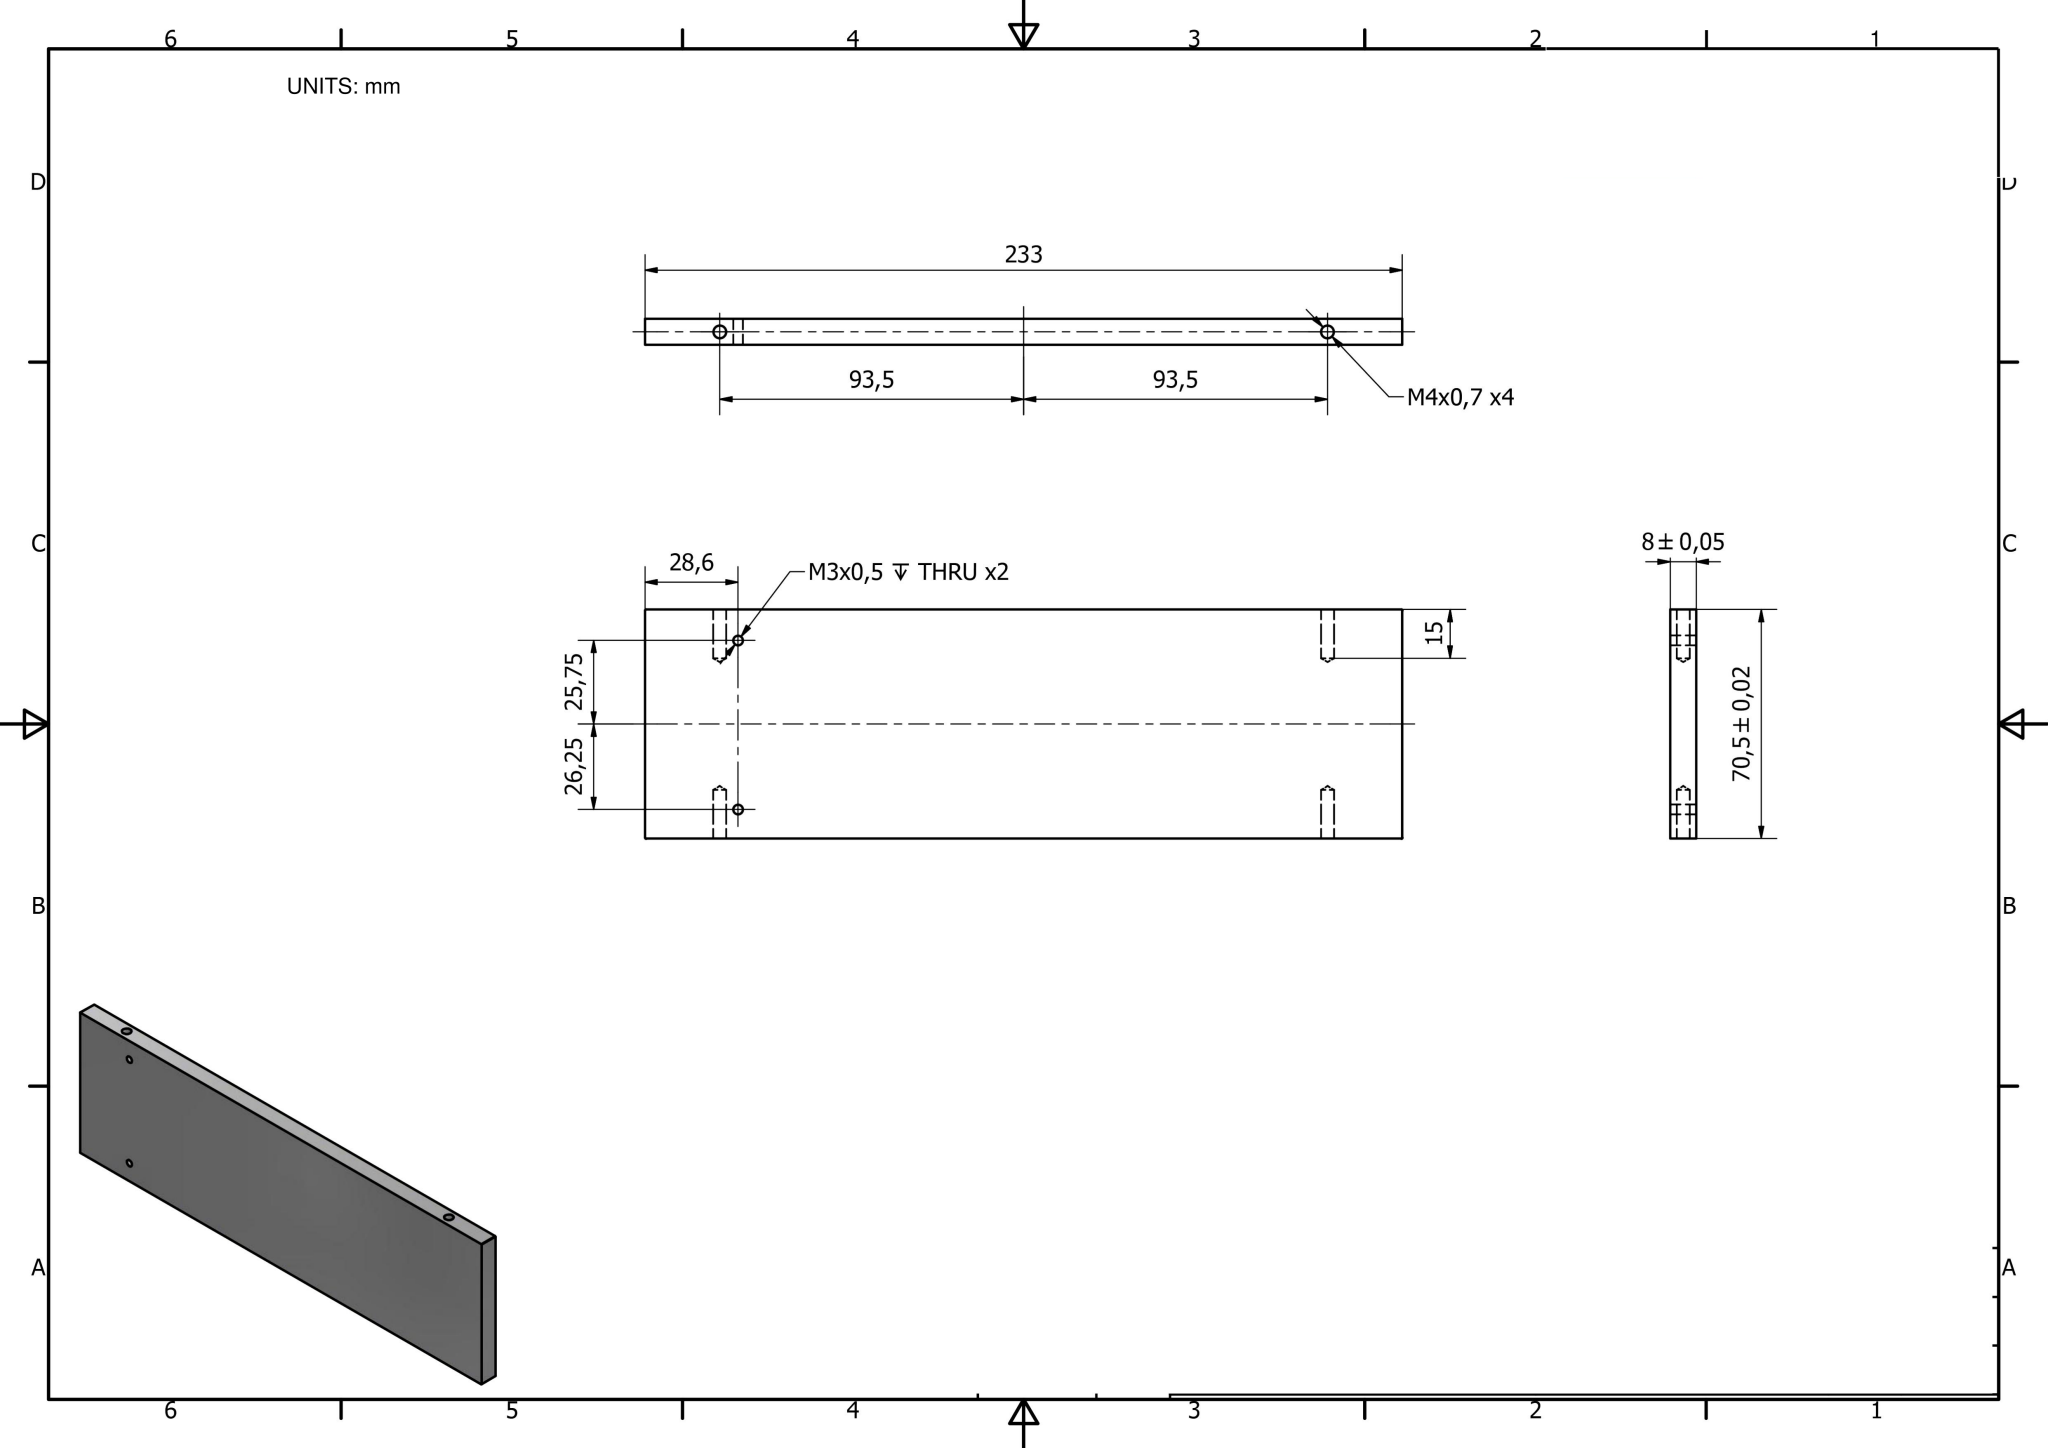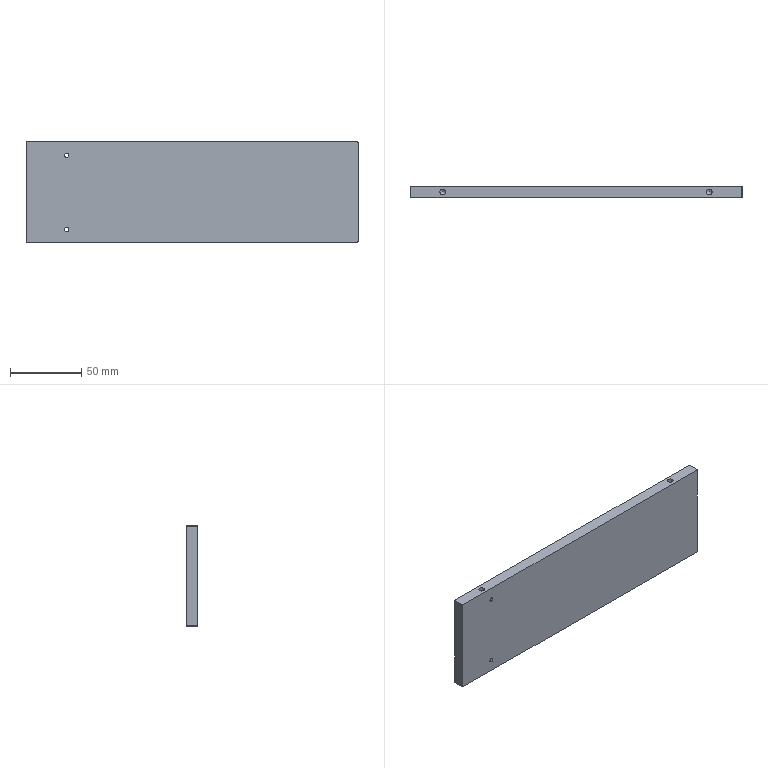Part | NX | mm | 1 solid | 20 faces | box 233 x 8 x 70.5 mm | volume 130524 mm3 | cylinder 10 | plane 6 | cone 4 | commonest cylinder face diameters 0.6 x4 4 x4 3 x2
STEP:
#1=DRAUGHTING_PRE_DEFINED_CURVE_FONT('');
#2=COLOUR_RGB('',0.9412,0.6275,0.4314);
#3=CURVE_STYLE('',#1,POSITIVE_LENGTH_MEASURE(0.000001),#2);
#4=PRESENTATION_STYLE_ASSIGNMENT((#3));
#5=CARTESIAN_POINT('',(389.001,-8.65,29.5));
#6=VERTEX_POINT('',#5);
#7=CARTESIAN_POINT('',(389.001,-6.65,29.5));
#8=DIRECTION('',(0.,0.,1.));
#9=DIRECTION('',(0.,1.,0.));
#10=AXIS2_PLACEMENT_3D('',#7,#8,#9);
#11=CIRCLE('',#10,2.);
#12=EDGE_CURVE('',#6,#6,#11,.T.);
#13=STYLED_ITEM('',(#4),#12);
#14=DRAUGHTING_PRE_DEFINED_CURVE_FONT('');
#15=COLOUR_RGB('',0.9412,0.6275,0.4314);
#16=CURVE_STYLE('',#14,POSITIVE_LENGTH_MEASURE(0.000001),#15);
#17=PRESENTATION_STYLE_ASSIGNMENT((#16));
#18=CARTESIAN_POINT('',(411.701,-10.65,29.5));
#19=VERTEX_POINT('',#18);
#20=CARTESIAN_POINT('',(411.701,-2.65,29.5));
#21=VERTEX_POINT('',#20);
#22=CARTESIAN_POINT('',(411.701,-10.65,29.5));
#23=DIRECTION('',(0.,1.,0.));
#24=VECTOR('',#23,1.);
#25=LINE('',#22,#24);
#26=EDGE_CURVE('',#19,#21,#25,.T.);
#27=STYLED_ITEM('',(#17),#26);
#28=COLOUR_RGB('',0.9412,0.6275,0.4314);
#29=FILL_AREA_STYLE_COLOUR('',#28);
#30=FILL_AREA_STYLE('',(#29));
#31=SURFACE_STYLE_FILL_AREA(#30);
#32=SURFACE_SIDE_STYLE('',(#31));
#33=SURFACE_STYLE_USAGE(.BOTH.,#32);
#34=PRESENTATION_STYLE_ASSIGNMENT((#33));
#35=CARTESIAN_POINT('',(412.001,-2.65,99.7));
#36=VERTEX_POINT('',#35);
#37=CARTESIAN_POINT('',(411.701,-2.65,100.));
#38=VERTEX_POINT('',#37);
#39=CARTESIAN_POINT('',(411.701,-2.65,99.7));
#40=DIRECTION('',(-0.,-1.,0.));
#41=DIRECTION('',(0.7071,0.,0.7071));
#42=AXIS2_PLACEMENT_3D('',#39,#40,#41);
#43=CIRCLE('',#42,0.3);
#44=EDGE_CURVE('',#36,#38,#43,.T.);
#45=ORIENTED_EDGE('',*,*,#44,.T.);
#46=CARTESIAN_POINT('',(411.701,-10.65,100.));
#47=VERTEX_POINT('',#46);
#48=CARTESIAN_POINT('',(411.701,-10.65,100.));
#49=DIRECTION('',(0.,-1.,0.));
#50=VECTOR('',#49,1.);
#51=LINE('',#48,#50);
#52=EDGE_CURVE('',#38,#47,#51,.T.);
#53=ORIENTED_EDGE('',*,*,#52,.T.);
#54=CARTESIAN_POINT('',(412.001,-10.65,99.7));
#55=VERTEX_POINT('',#54);
#56=CARTESIAN_POINT('',(411.701,-10.65,99.7));
#57=DIRECTION('',(0.,1.,-0.));
#58=DIRECTION('',(0.7071,0.,0.7071));
#59=AXIS2_PLACEMENT_3D('',#56,#57,#58);
#60=CIRCLE('',#59,0.3);
#61=EDGE_CURVE('',#47,#55,#60,.T.);
#62=ORIENTED_EDGE('',*,*,#61,.T.);
#63=CARTESIAN_POINT('',(412.001,-10.65,99.7));
#64=DIRECTION('',(0.,1.,0.));
#65=VECTOR('',#64,1.);
#66=LINE('',#63,#65);
#67=EDGE_CURVE('',#55,#36,#66,.T.);
#68=ORIENTED_EDGE('',*,*,#67,.T.);
#69=EDGE_LOOP('',(#45,#53,#62,#68));
#70=FACE_OUTER_BOUND('',#69,.T.);
#71=CARTESIAN_POINT('',(411.701,-10.65,99.7));
#72=DIRECTION('',(0.,1.,0.));
#73=DIRECTION('',(0.7071,0.,0.7071));
#74=AXIS2_PLACEMENT_3D('',#71,#72,#73);
#75=CYLINDRICAL_SURFACE('',#74,0.3);
#76=ADVANCED_FACE('',(#70),#75,.T.);
#77=CARTESIAN_POINT('',(207.601,-10.65,89.));
#78=VERTEX_POINT('',#77);
#79=CARTESIAN_POINT('',(207.601,-10.65,90.5));
#80=DIRECTION('',(-0.,-1.,0.));
#81=DIRECTION('',(0.,0.,1.));
#82=AXIS2_PLACEMENT_3D('',#79,#80,#81);
#83=CIRCLE('',#82,1.5);
#84=EDGE_CURVE('',#78,#78,#83,.F.);
#85=ORIENTED_EDGE('',*,*,#84,.T.);
#86=EDGE_LOOP('',(#85));
#87=FACE_BOUND('',#86,.T.);
#88=CARTESIAN_POINT('',(207.601,-10.65,37.));
#89=VERTEX_POINT('',#88);
#90=CARTESIAN_POINT('',(207.601,-10.65,38.5));
#91=DIRECTION('',(-0.,-1.,0.));
#92=DIRECTION('',(0.,0.,1.));
#93=AXIS2_PLACEMENT_3D('',#90,#91,#92);
#94=CIRCLE('',#93,1.5);
#95=EDGE_CURVE('',#89,#89,#94,.F.);
#96=ORIENTED_EDGE('',*,*,#95,.T.);
#97=EDGE_LOOP('',(#96));
#98=FACE_BOUND('',#97,.T.);
#99=ORIENTED_EDGE('',*,*,#61,.F.);
#100=CARTESIAN_POINT('',(179.301,-10.65,100.));
#101=VERTEX_POINT('',#100);
#102=CARTESIAN_POINT('',(179.001,-10.65,100.));
#103=DIRECTION('',(1.,0.,-0.));
#104=VECTOR('',#103,1.);
#105=LINE('',#102,#104);
#106=EDGE_CURVE('',#101,#47,#105,.T.);
#107=ORIENTED_EDGE('',*,*,#106,.F.);
#108=CARTESIAN_POINT('',(179.001,-10.65,99.7));
#109=VERTEX_POINT('',#108);
#110=CARTESIAN_POINT('',(179.301,-10.65,99.7));
#111=DIRECTION('',(0.,1.,-0.));
#112=DIRECTION('',(-0.7071,0.,0.7071));
#113=AXIS2_PLACEMENT_3D('',#110,#111,#112);
#114=CIRCLE('',#113,0.3);
#115=EDGE_CURVE('',#109,#101,#114,.T.);
#116=ORIENTED_EDGE('',*,*,#115,.F.);
#117=CARTESIAN_POINT('',(179.001,-10.65,29.8));
#118=VERTEX_POINT('',#117);
#119=CARTESIAN_POINT('',(179.001,-10.65,29.5));
#120=DIRECTION('',(0.,0.,1.));
#121=VECTOR('',#120,1.);
#122=LINE('',#119,#121);
#123=EDGE_CURVE('',#118,#109,#122,.T.);
#124=ORIENTED_EDGE('',*,*,#123,.F.);
#125=CARTESIAN_POINT('',(179.301,-10.65,29.5));
#126=VERTEX_POINT('',#125);
#127=CARTESIAN_POINT('',(179.301,-10.65,29.8));
#128=DIRECTION('',(0.,1.,-0.));
#129=DIRECTION('',(-0.7071,-0.,-0.7071));
#130=AXIS2_PLACEMENT_3D('',#127,#128,#129);
#131=CIRCLE('',#130,0.3);
#132=EDGE_CURVE('',#126,#118,#131,.T.);
#133=ORIENTED_EDGE('',*,*,#132,.F.);
#134=CARTESIAN_POINT('',(425.001,-10.65,29.5));
#135=DIRECTION('',(-1.,0.,0.));
#136=VECTOR('',#135,1.);
#137=LINE('',#134,#136);
#138=EDGE_CURVE('',#19,#126,#137,.T.);
#139=ORIENTED_EDGE('',*,*,#138,.F.);
#140=CARTESIAN_POINT('',(412.001,-10.65,29.8));
#141=VERTEX_POINT('',#140);
#142=CARTESIAN_POINT('',(411.701,-10.65,29.8));
#143=DIRECTION('',(0.,1.,-0.));
#144=DIRECTION('',(0.7071,-0.,-0.7071));
#145=AXIS2_PLACEMENT_3D('',#142,#143,#144);
#146=CIRCLE('',#145,0.3);
#147=EDGE_CURVE('',#141,#19,#146,.T.);
#148=ORIENTED_EDGE('',*,*,#147,.F.);
#149=CARTESIAN_POINT('',(412.001,-10.65,64.75));
#150=DIRECTION('',(0.,0.,1.));
#151=VECTOR('',#150,1.);
#152=LINE('',#149,#151);
#153=EDGE_CURVE('',#55,#141,#152,.F.);
#154=ORIENTED_EDGE('',*,*,#153,.F.);
#155=EDGE_LOOP('',(#99,#107,#116,#124,#133,#139,#148,#154));
#156=FACE_OUTER_BOUND('',#155,.T.);
#157=CARTESIAN_POINT('',(302.001,-10.65,64.75));
#158=DIRECTION('',(0.,1.,-0.));
#159=DIRECTION('',(0.,0.,1.));
#160=AXIS2_PLACEMENT_3D('',#157,#158,#159);
#161=PLANE('',#160);
#162=ADVANCED_FACE('',(#87,#98,#156),#161,.F.);
#163=CARTESIAN_POINT('',(389.001,-4.65,100.));
#164=VERTEX_POINT('',#163);
#165=CARTESIAN_POINT('',(389.001,-6.65,100.));
#166=DIRECTION('',(-0.,0.,-1.));
#167=DIRECTION('',(0.,-1.,0.));
#168=AXIS2_PLACEMENT_3D('',#165,#166,#167);
#169=CIRCLE('',#168,2.);
#170=EDGE_CURVE('',#164,#164,#169,.T.);
#171=ORIENTED_EDGE('',*,*,#170,.T.);
#172=EDGE_LOOP('',(#171));
#173=FACE_BOUND('',#172,.T.);
#174=CARTESIAN_POINT('',(202.001,-4.65,100.));
#175=VERTEX_POINT('',#174);
#176=CARTESIAN_POINT('',(202.001,-6.65,100.));
#177=DIRECTION('',(-0.,0.,-1.));
#178=DIRECTION('',(0.,-1.,0.));
#179=AXIS2_PLACEMENT_3D('',#176,#177,#178);
#180=CIRCLE('',#179,2.);
#181=EDGE_CURVE('',#175,#175,#180,.T.);
#182=ORIENTED_EDGE('',*,*,#181,.T.);
#183=EDGE_LOOP('',(#182));
#184=FACE_BOUND('',#183,.T.);
#185=ORIENTED_EDGE('',*,*,#52,.F.);
#186=CARTESIAN_POINT('',(179.301,-2.65,100.));
#187=VERTEX_POINT('',#186);
#188=CARTESIAN_POINT('',(179.001,-2.65,100.));
#189=DIRECTION('',(-1.,0.,0.));
#190=VECTOR('',#189,1.);
#191=LINE('',#188,#190);
#192=EDGE_CURVE('',#38,#187,#191,.T.);
#193=ORIENTED_EDGE('',*,*,#192,.T.);
#194=CARTESIAN_POINT('',(179.301,-10.65,100.));
#195=DIRECTION('',(0.,1.,0.));
#196=VECTOR('',#195,1.);
#197=LINE('',#194,#196);
#198=EDGE_CURVE('',#101,#187,#197,.T.);
#199=ORIENTED_EDGE('',*,*,#198,.F.);
#200=ORIENTED_EDGE('',*,*,#106,.T.);
#201=EDGE_LOOP('',(#185,#193,#199,#200));
#202=FACE_OUTER_BOUND('',#201,.T.);
#203=CARTESIAN_POINT('',(302.001,-10.65,100.));
#204=DIRECTION('',(0.,0.,1.));
#205=DIRECTION('',(1.,0.,-0.));
#206=AXIS2_PLACEMENT_3D('',#203,#204,#205);
#207=PLANE('',#206);
#208=ADVANCED_FACE('',(#173,#184,#202),#207,.T.);
#209=CARTESIAN_POINT('',(179.001,-2.65,99.7));
#210=VERTEX_POINT('',#209);
#211=CARTESIAN_POINT('',(179.301,-2.65,99.7));
#212=DIRECTION('',(-0.,-1.,0.));
#213=DIRECTION('',(-0.7071,0.,0.7071));
#214=AXIS2_PLACEMENT_3D('',#211,#212,#213);
#215=CIRCLE('',#214,0.3);
#216=EDGE_CURVE('',#187,#210,#215,.T.);
#217=ORIENTED_EDGE('',*,*,#216,.T.);
#218=CARTESIAN_POINT('',(179.001,-10.65,99.7));
#219=DIRECTION('',(0.,-1.,0.));
#220=VECTOR('',#219,1.);
#221=LINE('',#218,#220);
#222=EDGE_CURVE('',#210,#109,#221,.T.);
#223=ORIENTED_EDGE('',*,*,#222,.T.);
#224=ORIENTED_EDGE('',*,*,#115,.T.);
#225=ORIENTED_EDGE('',*,*,#198,.T.);
#226=EDGE_LOOP('',(#217,#223,#224,#225));
#227=FACE_OUTER_BOUND('',#226,.T.);
#228=CARTESIAN_POINT('',(179.301,-10.65,99.7));
#229=DIRECTION('',(0.,1.,0.));
#230=DIRECTION('',(-0.7071,0.,0.7071));
#231=AXIS2_PLACEMENT_3D('',#228,#229,#230);
#232=CYLINDRICAL_SURFACE('',#231,0.3);
#233=ADVANCED_FACE('',(#227),#232,.T.);
#234=CARTESIAN_POINT('',(412.001,-2.65,29.8));
#235=VERTEX_POINT('',#234);
#236=CARTESIAN_POINT('',(411.701,-2.65,29.8));
#237=DIRECTION('',(-0.,-1.,0.));
#238=DIRECTION('',(0.7071,-0.,-0.7071));
#239=AXIS2_PLACEMENT_3D('',#236,#237,#238);
#240=CIRCLE('',#239,0.3);
#241=EDGE_CURVE('',#21,#235,#240,.T.);
#242=ORIENTED_EDGE('',*,*,#241,.T.);
#243=CARTESIAN_POINT('',(412.001,-10.65,29.8));
#244=DIRECTION('',(0.,-1.,0.));
#245=VECTOR('',#244,1.);
#246=LINE('',#243,#245);
#247=EDGE_CURVE('',#235,#141,#246,.T.);
#248=ORIENTED_EDGE('',*,*,#247,.T.);
#249=ORIENTED_EDGE('',*,*,#147,.T.);
#250=ORIENTED_EDGE('',*,*,#26,.T.);
#251=EDGE_LOOP('',(#242,#248,#249,#250));
#252=FACE_OUTER_BOUND('',#251,.T.);
#253=CARTESIAN_POINT('',(411.701,-10.65,29.8));
#254=DIRECTION('',(0.,1.,0.));
#255=DIRECTION('',(0.7071,0.,-0.7071));
#256=AXIS2_PLACEMENT_3D('',#253,#254,#255);
#257=CYLINDRICAL_SURFACE('',#256,0.3);
#258=ADVANCED_FACE('',(#252),#257,.T.);
#259=CARTESIAN_POINT('',(202.001,-8.65,29.5));
#260=VERTEX_POINT('',#259);
#261=CARTESIAN_POINT('',(202.001,-6.65,29.5));
#262=DIRECTION('',(0.,0.,1.));
#263=DIRECTION('',(0.,1.,0.));
#264=AXIS2_PLACEMENT_3D('',#261,#262,#263);
#265=CIRCLE('',#264,2.);
#266=EDGE_CURVE('',#260,#260,#265,.T.);
#267=ORIENTED_EDGE('',*,*,#266,.T.);
#268=EDGE_LOOP('',(#267));
#269=FACE_BOUND('',#268,.T.);
#270=ORIENTED_EDGE('',*,*,#12,.T.);
#271=EDGE_LOOP('',(#270));
#272=FACE_BOUND('',#271,.T.);
#273=ORIENTED_EDGE('',*,*,#26,.F.);
#274=ORIENTED_EDGE('',*,*,#138,.T.);
#275=CARTESIAN_POINT('',(179.301,-2.65,29.5));
#276=VERTEX_POINT('',#275);
#277=CARTESIAN_POINT('',(179.301,-10.65,29.5));
#278=DIRECTION('',(0.,-1.,0.));
#279=VECTOR('',#278,1.);
#280=LINE('',#277,#279);
#281=EDGE_CURVE('',#276,#126,#280,.T.);
#282=ORIENTED_EDGE('',*,*,#281,.F.);
#283=CARTESIAN_POINT('',(425.001,-2.65,29.5));
#284=DIRECTION('',(1.,0.,-0.));
#285=VECTOR('',#284,1.);
#286=LINE('',#283,#285);
#287=EDGE_CURVE('',#276,#21,#286,.T.);
#288=ORIENTED_EDGE('',*,*,#287,.T.);
#289=EDGE_LOOP('',(#273,#274,#282,#288));
#290=FACE_OUTER_BOUND('',#289,.T.);
#291=CARTESIAN_POINT('',(302.001,-10.65,29.5));
#292=DIRECTION('',(-0.,0.,-1.));
#293=DIRECTION('',(-1.,0.,0.));
#294=AXIS2_PLACEMENT_3D('',#291,#292,#293);
#295=PLANE('',#294);
#296=ADVANCED_FACE('',(#269,#272,#290),#295,.T.);
#297=CARTESIAN_POINT('',(179.001,-2.65,29.8));
#298=VERTEX_POINT('',#297);
#299=CARTESIAN_POINT('',(179.301,-2.65,29.8));
#300=DIRECTION('',(-0.,-1.,0.));
#301=DIRECTION('',(-0.7071,-0.,-0.7071));
#302=AXIS2_PLACEMENT_3D('',#299,#300,#301);
#303=CIRCLE('',#302,0.3);
#304=EDGE_CURVE('',#298,#276,#303,.T.);
#305=ORIENTED_EDGE('',*,*,#304,.T.);
#306=ORIENTED_EDGE('',*,*,#281,.T.);
#307=ORIENTED_EDGE('',*,*,#132,.T.);
#308=CARTESIAN_POINT('',(179.001,-10.65,29.8));
#309=DIRECTION('',(0.,1.,0.));
#310=VECTOR('',#309,1.);
#311=LINE('',#308,#310);
#312=EDGE_CURVE('',#118,#298,#311,.T.);
#313=ORIENTED_EDGE('',*,*,#312,.T.);
#314=EDGE_LOOP('',(#305,#306,#307,#313));
#315=FACE_OUTER_BOUND('',#314,.T.);
#316=CARTESIAN_POINT('',(179.301,-10.65,29.8));
#317=DIRECTION('',(0.,1.,0.));
#318=DIRECTION('',(-0.7071,0.,-0.7071));
#319=AXIS2_PLACEMENT_3D('',#316,#317,#318);
#320=CYLINDRICAL_SURFACE('',#319,0.3);
#321=ADVANCED_FACE('',(#315),#320,.T.);
#322=ORIENTED_EDGE('',*,*,#67,.F.);
#323=ORIENTED_EDGE('',*,*,#153,.T.);
#324=ORIENTED_EDGE('',*,*,#247,.F.);
#325=CARTESIAN_POINT('',(412.001,-2.65,64.75));
#326=DIRECTION('',(0.,0.,1.));
#327=VECTOR('',#326,1.);
#328=LINE('',#325,#327);
#329=EDGE_CURVE('',#235,#36,#328,.T.);
#330=ORIENTED_EDGE('',*,*,#329,.T.);
#331=EDGE_LOOP('',(#322,#323,#324,#330));
#332=FACE_OUTER_BOUND('',#331,.T.);
#333=CARTESIAN_POINT('',(412.001,-10.65,64.75));
#334=DIRECTION('',(1.,0.,0.));
#335=DIRECTION('',(0.,0.,-1.));
#336=AXIS2_PLACEMENT_3D('',#333,#334,#335);
#337=PLANE('',#336);
#338=ADVANCED_FACE('',(#332),#337,.T.);
#339=ORIENTED_EDGE('',*,*,#44,.F.);
#340=ORIENTED_EDGE('',*,*,#329,.F.);
#341=ORIENTED_EDGE('',*,*,#241,.F.);
#342=ORIENTED_EDGE('',*,*,#287,.F.);
#343=ORIENTED_EDGE('',*,*,#304,.F.);
#344=CARTESIAN_POINT('',(179.001,-2.65,29.5));
#345=DIRECTION('',(0.,0.,-1.));
#346=VECTOR('',#345,1.);
#347=LINE('',#344,#346);
#348=EDGE_CURVE('',#210,#298,#347,.T.);
#349=ORIENTED_EDGE('',*,*,#348,.F.);
#350=ORIENTED_EDGE('',*,*,#216,.F.);
#351=ORIENTED_EDGE('',*,*,#192,.F.);
#352=EDGE_LOOP('',(#339,#340,#341,#342,#343,#349,#350,#351));
#353=FACE_OUTER_BOUND('',#352,.T.);
#354=CARTESIAN_POINT('',(207.601,-2.65,89.));
#355=VERTEX_POINT('',#354);
#356=CARTESIAN_POINT('',(207.601,-2.65,90.5));
#357=DIRECTION('',(-0.,-1.,0.));
#358=DIRECTION('',(0.,0.,1.));
#359=AXIS2_PLACEMENT_3D('',#356,#357,#358);
#360=CIRCLE('',#359,1.5);
#361=EDGE_CURVE('',#355,#355,#360,.T.);
#362=ORIENTED_EDGE('',*,*,#361,.T.);
#363=EDGE_LOOP('',(#362));
#364=FACE_BOUND('',#363,.T.);
#365=CARTESIAN_POINT('',(207.601,-2.65,37.));
#366=VERTEX_POINT('',#365);
#367=CARTESIAN_POINT('',(207.601,-2.65,38.5));
#368=DIRECTION('',(-0.,-1.,0.));
#369=DIRECTION('',(0.,0.,1.));
#370=AXIS2_PLACEMENT_3D('',#367,#368,#369);
#371=CIRCLE('',#370,1.5);
#372=EDGE_CURVE('',#366,#366,#371,.T.);
#373=ORIENTED_EDGE('',*,*,#372,.T.);
#374=EDGE_LOOP('',(#373));
#375=FACE_BOUND('',#374,.T.);
#376=CARTESIAN_POINT('',(302.001,-2.65,64.75));
#377=DIRECTION('',(0.,1.,-0.));
#378=DIRECTION('',(0.,0.,1.));
#379=AXIS2_PLACEMENT_3D('',#376,#377,#378);
#380=PLANE('',#379);
#381=ADVANCED_FACE('',(#353,#364,#375),#380,.T.);
#382=CARTESIAN_POINT('',(389.001,-8.65,85.));
#383=VERTEX_POINT('',#382);
#384=CARTESIAN_POINT('',(389.001,-6.65,85.));
#385=DIRECTION('',(0.,0.,1.));
#386=DIRECTION('',(0.,-1.,0.));
#387=AXIS2_PLACEMENT_3D('',#384,#385,#386);
#388=CIRCLE('',#387,2.);
#389=EDGE_CURVE('',#383,#383,#388,.T.);
#390=ORIENTED_EDGE('',*,*,#389,.T.);
#391=EDGE_LOOP('',(#390));
#392=FACE_BOUND('',#391,.T.);
#393=CARTESIAN_POINT('',(389.001,-6.65,83.798));
#394=VERTEX_POINT('',#393);
#395=VERTEX_LOOP('',#394);
#396=FACE_BOUND('',#395,.T.);
#397=CARTESIAN_POINT('',(389.001,-6.65,84.399));
#398=DIRECTION('',(0.,0.,1.));
#399=DIRECTION('',(1.,0.,0.));
#400=AXIS2_PLACEMENT_3D('',#397,#398,#399);
#401=CONICAL_SURFACE('',#400,1.,1.03);
#402=ADVANCED_FACE('',(#392,#396),#401,.F.);
#403=ORIENTED_EDGE('',*,*,#170,.F.);
#404=EDGE_LOOP('',(#403));
#405=FACE_BOUND('',#404,.T.);
#406=ORIENTED_EDGE('',*,*,#389,.F.);
#407=EDGE_LOOP('',(#406));
#408=FACE_BOUND('',#407,.T.);
#409=CARTESIAN_POINT('',(389.001,-6.65,104.));
#410=DIRECTION('',(0.,0.,-1.));
#411=DIRECTION('',(0.,-1.,0.));
#412=AXIS2_PLACEMENT_3D('',#409,#410,#411);
#413=CYLINDRICAL_SURFACE('',#412,2.);
#414=ADVANCED_FACE('',(#405,#408),#413,.F.);
#415=CARTESIAN_POINT('',(202.001,-8.65,85.));
#416=VERTEX_POINT('',#415);
#417=CARTESIAN_POINT('',(202.001,-6.65,85.));
#418=DIRECTION('',(0.,0.,1.));
#419=DIRECTION('',(0.,-1.,0.));
#420=AXIS2_PLACEMENT_3D('',#417,#418,#419);
#421=CIRCLE('',#420,2.);
#422=EDGE_CURVE('',#416,#416,#421,.T.);
#423=ORIENTED_EDGE('',*,*,#422,.T.);
#424=EDGE_LOOP('',(#423));
#425=FACE_BOUND('',#424,.T.);
#426=CARTESIAN_POINT('',(202.001,-6.65,83.798));
#427=VERTEX_POINT('',#426);
#428=VERTEX_LOOP('',#427);
#429=FACE_BOUND('',#428,.T.);
#430=CARTESIAN_POINT('',(202.001,-6.65,84.399));
#431=DIRECTION('',(0.,0.,1.));
#432=DIRECTION('',(1.,0.,0.));
#433=AXIS2_PLACEMENT_3D('',#430,#431,#432);
#434=CONICAL_SURFACE('',#433,1.,1.03);
#435=ADVANCED_FACE('',(#425,#429),#434,.F.);
#436=ORIENTED_EDGE('',*,*,#181,.F.);
#437=EDGE_LOOP('',(#436));
#438=FACE_BOUND('',#437,.T.);
#439=ORIENTED_EDGE('',*,*,#422,.F.);
#440=EDGE_LOOP('',(#439));
#441=FACE_BOUND('',#440,.T.);
#442=CARTESIAN_POINT('',(202.001,-6.65,104.));
#443=DIRECTION('',(0.,0.,-1.));
#444=DIRECTION('',(0.,-1.,0.));
#445=AXIS2_PLACEMENT_3D('',#442,#443,#444);
#446=CYLINDRICAL_SURFACE('',#445,2.);
#447=ADVANCED_FACE('',(#438,#441),#446,.F.);
#448=CARTESIAN_POINT('',(202.001,-4.65,44.5));
#449=VERTEX_POINT('',#448);
#450=CARTESIAN_POINT('',(202.001,-6.65,44.5));
#451=DIRECTION('',(-0.,0.,-1.));
#452=DIRECTION('',(0.,1.,0.));
#453=AXIS2_PLACEMENT_3D('',#450,#451,#452);
#454=CIRCLE('',#453,2.);
#455=EDGE_CURVE('',#449,#449,#454,.T.);
#456=ORIENTED_EDGE('',*,*,#455,.T.);
#457=EDGE_LOOP('',(#456));
#458=FACE_BOUND('',#457,.T.);
#459=CARTESIAN_POINT('',(202.001,-6.65,45.702));
#460=VERTEX_POINT('',#459);
#461=VERTEX_LOOP('',#460);
#462=FACE_BOUND('',#461,.T.);
#463=CARTESIAN_POINT('',(202.001,-6.65,45.101));
#464=DIRECTION('',(0.,0.,-1.));
#465=DIRECTION('',(1.,0.,0.));
#466=AXIS2_PLACEMENT_3D('',#463,#464,#465);
#467=CONICAL_SURFACE('',#466,1.,1.03);
#468=ADVANCED_FACE('',(#458,#462),#467,.F.);
#469=ORIENTED_EDGE('',*,*,#266,.F.);
#470=EDGE_LOOP('',(#469));
#471=FACE_BOUND('',#470,.T.);
#472=ORIENTED_EDGE('',*,*,#455,.F.);
#473=EDGE_LOOP('',(#472));
#474=FACE_BOUND('',#473,.T.);
#475=CARTESIAN_POINT('',(202.001,-6.65,25.5));
#476=DIRECTION('',(0.,0.,1.));
#477=DIRECTION('',(0.,1.,0.));
#478=AXIS2_PLACEMENT_3D('',#475,#476,#477);
#479=CYLINDRICAL_SURFACE('',#478,2.);
#480=ADVANCED_FACE('',(#471,#474),#479,.F.);
#481=CARTESIAN_POINT('',(389.001,-4.65,44.5));
#482=VERTEX_POINT('',#481);
#483=CARTESIAN_POINT('',(389.001,-6.65,44.5));
#484=DIRECTION('',(-0.,0.,-1.));
#485=DIRECTION('',(0.,1.,0.));
#486=AXIS2_PLACEMENT_3D('',#483,#484,#485);
#487=CIRCLE('',#486,2.);
#488=EDGE_CURVE('',#482,#482,#487,.T.);
#489=ORIENTED_EDGE('',*,*,#488,.T.);
#490=EDGE_LOOP('',(#489));
#491=FACE_BOUND('',#490,.T.);
#492=CARTESIAN_POINT('',(389.001,-6.65,45.702));
#493=VERTEX_POINT('',#492);
#494=VERTEX_LOOP('',#493);
#495=FACE_BOUND('',#494,.T.);
#496=CARTESIAN_POINT('',(389.001,-6.65,45.101));
#497=DIRECTION('',(0.,0.,-1.));
#498=DIRECTION('',(1.,0.,0.));
#499=AXIS2_PLACEMENT_3D('',#496,#497,#498);
#500=CONICAL_SURFACE('',#499,1.,1.03);
#501=ADVANCED_FACE('',(#491,#495),#500,.F.);
#502=ORIENTED_EDGE('',*,*,#12,.F.);
#503=EDGE_LOOP('',(#502));
#504=FACE_BOUND('',#503,.T.);
#505=ORIENTED_EDGE('',*,*,#488,.F.);
#506=EDGE_LOOP('',(#505));
#507=FACE_BOUND('',#506,.T.);
#508=CARTESIAN_POINT('',(389.001,-6.65,25.5));
#509=DIRECTION('',(0.,0.,1.));
#510=DIRECTION('',(0.,1.,0.));
#511=AXIS2_PLACEMENT_3D('',#508,#509,#510);
#512=CYLINDRICAL_SURFACE('',#511,2.);
#513=ADVANCED_FACE('',(#504,#507),#512,.F.);
#514=ORIENTED_EDGE('',*,*,#84,.F.);
#515=EDGE_LOOP('',(#514));
#516=FACE_BOUND('',#515,.T.);
#517=ORIENTED_EDGE('',*,*,#361,.F.);
#518=EDGE_LOOP('',(#517));
#519=FACE_BOUND('',#518,.T.);
#520=CARTESIAN_POINT('',(207.601,0.35,90.5));
#521=DIRECTION('',(0.,-1.,0.));
#522=DIRECTION('',(0.,0.,1.));
#523=AXIS2_PLACEMENT_3D('',#520,#521,#522);
#524=CYLINDRICAL_SURFACE('',#523,1.5);
#525=ADVANCED_FACE('',(#516,#519),#524,.F.);
#526=ORIENTED_EDGE('',*,*,#95,.F.);
#527=EDGE_LOOP('',(#526));
#528=FACE_BOUND('',#527,.T.);
#529=ORIENTED_EDGE('',*,*,#372,.F.);
#530=EDGE_LOOP('',(#529));
#531=FACE_BOUND('',#530,.T.);
#532=CARTESIAN_POINT('',(207.601,0.35,38.5));
#533=DIRECTION('',(0.,-1.,0.));
#534=DIRECTION('',(0.,0.,1.));
#535=AXIS2_PLACEMENT_3D('',#532,#533,#534);
#536=CYLINDRICAL_SURFACE('',#535,1.5);
#537=ADVANCED_FACE('',(#528,#531),#536,.F.);
#538=ORIENTED_EDGE('',*,*,#222,.F.);
#539=ORIENTED_EDGE('',*,*,#348,.T.);
#540=ORIENTED_EDGE('',*,*,#312,.F.);
#541=ORIENTED_EDGE('',*,*,#123,.T.);
#542=EDGE_LOOP('',(#538,#539,#540,#541));
#543=FACE_OUTER_BOUND('',#542,.T.);
#544=CARTESIAN_POINT('',(179.001,-10.65,64.75));
#545=DIRECTION('',(-1.,0.,0.));
#546=DIRECTION('',(0.,0.,1.));
#547=AXIS2_PLACEMENT_3D('',#544,#545,#546);
#548=PLANE('',#547);
#549=ADVANCED_FACE('',(#543),#548,.T.);
#550=CLOSED_SHELL('',(#76,#162,#208,#233,#258,#296,#321,#338,#381,#402,#414,#435,#447,#468,#480,#501,#513,#525,#537,#549));
#551=MANIFOLD_SOLID_BREP('',#550);
#552=STYLED_ITEM('',(#34),#551);
#553=DRAUGHTING_PRE_DEFINED_CURVE_FONT('');
#554=COLOUR_RGB('',0.9412,0.6275,0.4314);
#555=CURVE_STYLE('',#553,POSITIVE_LENGTH_MEASURE(0.000001),#554);
#556=PRESENTATION_STYLE_ASSIGNMENT((#555));
#557=STYLED_ITEM('',(#556),#198);
#558=COLOUR_RGB('',0.9412,0.6275,0.4314);
#559=FILL_AREA_STYLE_COLOUR('',#558);
#560=FILL_AREA_STYLE('',(#559));
#561=SURFACE_STYLE_FILL_AREA(#560);
#562=SURFACE_SIDE_STYLE('',(#561));
#563=SURFACE_STYLE_USAGE(.BOTH.,#562);
#564=PRESENTATION_STYLE_ASSIGNMENT((#563));
#565=STYLED_ITEM('',(#564),#501);
#566=COLOUR_RGB('',0.9412,0.6275,0.4314);
#567=FILL_AREA_STYLE_COLOUR('',#566);
#568=FILL_AREA_STYLE('',(#567));
#569=SURFACE_STYLE_FILL_AREA(#568);
#570=SURFACE_SIDE_STYLE('',(#569));
#571=SURFACE_STYLE_USAGE(.BOTH.,#570);
#572=PRESENTATION_STYLE_ASSIGNMENT((#571));
#573=STYLED_ITEM('',(#572),#208);
#574=DRAUGHTING_PRE_DEFINED_CURVE_FONT('');
#575=COLOUR_RGB('',0.9412,0.6275,0.4314);
#576=CURVE_STYLE('',#574,POSITIVE_LENGTH_MEASURE(0.000001),#575);
#577=PRESENTATION_STYLE_ASSIGNMENT((#576));
#578=STYLED_ITEM('',(#577),#372);
#579=COLOUR_RGB('',0.9412,0.6275,0.4314);
#580=FILL_AREA_STYLE_COLOUR('',#579);
#581=FILL_AREA_STYLE('',(#580));
#582=SURFACE_STYLE_FILL_AREA(#581);
#583=SURFACE_SIDE_STYLE('',(#582));
#584=SURFACE_STYLE_USAGE(.BOTH.,#583);
#585=PRESENTATION_STYLE_ASSIGNMENT((#584));
#586=STYLED_ITEM('',(#585),#321);
#587=COLOUR_RGB('',0.9412,0.6275,0.4314);
#588=FILL_AREA_STYLE_COLOUR('',#587);
#589=FILL_AREA_STYLE('',(#588));
#590=SURFACE_STYLE_FILL_AREA(#589);
#591=SURFACE_SIDE_STYLE('',(#590));
#592=SURFACE_STYLE_USAGE(.BOTH.,#591);
#593=PRESENTATION_STYLE_ASSIGNMENT((#592));
#594=STYLED_ITEM('',(#593),#537);
#595=COLOUR_RGB('',0.9412,0.6275,0.4314);
#596=FILL_AREA_STYLE_COLOUR('',#595);
#597=FILL_AREA_STYLE('',(#596));
#598=SURFACE_STYLE_FILL_AREA(#597);
#599=SURFACE_SIDE_STYLE('',(#598));
#600=SURFACE_STYLE_USAGE(.BOTH.,#599);
#601=PRESENTATION_STYLE_ASSIGNMENT((#600));
#602=STYLED_ITEM('',(#601),#525);
#603=COLOUR_RGB('',0.9412,0.6275,0.4314);
#604=FILL_AREA_STYLE_COLOUR('',#603);
#605=FILL_AREA_STYLE('',(#604));
#606=SURFACE_STYLE_FILL_AREA(#605);
#607=SURFACE_SIDE_STYLE('',(#606));
#608=SURFACE_STYLE_USAGE(.BOTH.,#607);
#609=PRESENTATION_STYLE_ASSIGNMENT((#608));
#610=STYLED_ITEM('',(#609),#338);
#611=COLOUR_RGB('',0.9412,0.6275,0.4314);
#612=FILL_AREA_STYLE_COLOUR('',#611);
#613=FILL_AREA_STYLE('',(#612));
#614=SURFACE_STYLE_FILL_AREA(#613);
#615=SURFACE_SIDE_STYLE('',(#614));
#616=SURFACE_STYLE_USAGE(.BOTH.,#615);
#617=PRESENTATION_STYLE_ASSIGNMENT((#616));
#618=STYLED_ITEM('',(#617),#447);
#619=COLOUR_RGB('',0.9412,0.6275,0.4314);
#620=FILL_AREA_STYLE_COLOUR('',#619);
#621=FILL_AREA_STYLE('',(#620));
#622=SURFACE_STYLE_FILL_AREA(#621);
#623=SURFACE_SIDE_STYLE('',(#622));
#624=SURFACE_STYLE_USAGE(.BOTH.,#623);
#625=PRESENTATION_STYLE_ASSIGNMENT((#624));
#626=STYLED_ITEM('',(#625),#414);
#627=DRAUGHTING_PRE_DEFINED_CURVE_FONT('');
#628=COLOUR_RGB('',0.9412,0.6275,0.4314);
#629=CURVE_STYLE('',#627,POSITIVE_LENGTH_MEASURE(0.000001),#628);
#630=PRESENTATION_STYLE_ASSIGNMENT((#629));
#631=STYLED_ITEM('',(#630),#348);
#632=DRAUGHTING_PRE_DEFINED_CURVE_FONT('');
#633=COLOUR_RGB('',0.9412,0.6275,0.4314);
#634=CURVE_STYLE('',#632,POSITIVE_LENGTH_MEASURE(0.000001),#633);
#635=PRESENTATION_STYLE_ASSIGNMENT((#634));
#636=STYLED_ITEM('',(#635),#488);
#637=DRAUGHTING_PRE_DEFINED_CURVE_FONT('');
#638=COLOUR_RGB('',0.9412,0.6275,0.4314);
#639=CURVE_STYLE('',#637,POSITIVE_LENGTH_MEASURE(0.000001),#638);
#640=PRESENTATION_STYLE_ASSIGNMENT((#639));
#641=STYLED_ITEM('',(#640),#84);
#642=DRAUGHTING_PRE_DEFINED_CURVE_FONT('');
#643=COLOUR_RGB('',0.9412,0.6275,0.4314);
#644=CURVE_STYLE('',#642,POSITIVE_LENGTH_MEASURE(0.000001),#643);
#645=PRESENTATION_STYLE_ASSIGNMENT((#644));
#646=STYLED_ITEM('',(#645),#44);
#647=COLOUR_RGB('',0.9412,0.6275,0.4314);
#648=FILL_AREA_STYLE_COLOUR('',#647);
#649=FILL_AREA_STYLE('',(#648));
#650=SURFACE_STYLE_FILL_AREA(#649);
#651=SURFACE_SIDE_STYLE('',(#650));
#652=SURFACE_STYLE_USAGE(.BOTH.,#651);
#653=PRESENTATION_STYLE_ASSIGNMENT((#652));
#654=STYLED_ITEM('',(#653),#513);
#655=COLOUR_RGB('',0.9412,0.6275,0.4314);
#656=FILL_AREA_STYLE_COLOUR('',#655);
#657=FILL_AREA_STYLE('',(#656));
#658=SURFACE_STYLE_FILL_AREA(#657);
#659=SURFACE_SIDE_STYLE('',(#658));
#660=SURFACE_STYLE_USAGE(.BOTH.,#659);
#661=PRESENTATION_STYLE_ASSIGNMENT((#660));
#662=STYLED_ITEM('',(#661),#233);
#663=DRAUGHTING_PRE_DEFINED_CURVE_FONT('');
#664=COLOUR_RGB('',0.9412,0.6275,0.4314);
#665=CURVE_STYLE('',#663,POSITIVE_LENGTH_MEASURE(0.000001),#664);
#666=PRESENTATION_STYLE_ASSIGNMENT((#665));
#667=STYLED_ITEM('',(#666),#138);
#668=DRAUGHTING_PRE_DEFINED_CURVE_FONT('');
#669=COLOUR_RGB('',0.9412,0.6275,0.4314);
#670=CURVE_STYLE('',#668,POSITIVE_LENGTH_MEASURE(0.000001),#669);
#671=PRESENTATION_STYLE_ASSIGNMENT((#670));
#672=STYLED_ITEM('',(#671),#312);
#673=DRAUGHTING_PRE_DEFINED_CURVE_FONT('');
#674=COLOUR_RGB('',0.9412,0.6275,0.4314);
#675=CURVE_STYLE('',#673,POSITIVE_LENGTH_MEASURE(0.000001),#674);
#676=PRESENTATION_STYLE_ASSIGNMENT((#675));
#677=STYLED_ITEM('',(#676),#329);
#678=DRAUGHTING_PRE_DEFINED_CURVE_FONT('');
#679=COLOUR_RGB('',0.9412,0.6275,0.4314);
#680=CURVE_STYLE('',#678,POSITIVE_LENGTH_MEASURE(0.000001),#679);
#681=PRESENTATION_STYLE_ASSIGNMENT((#680));
#682=STYLED_ITEM('',(#681),#455);
#683=COLOUR_RGB('',0.9412,0.6275,0.4314);
#684=FILL_AREA_STYLE_COLOUR('',#683);
#685=FILL_AREA_STYLE('',(#684));
#686=SURFACE_STYLE_FILL_AREA(#685);
#687=SURFACE_SIDE_STYLE('',(#686));
#688=SURFACE_STYLE_USAGE(.BOTH.,#687);
#689=PRESENTATION_STYLE_ASSIGNMENT((#688));
#690=STYLED_ITEM('',(#689),#258);
#691=DRAUGHTING_PRE_DEFINED_CURVE_FONT('');
#692=COLOUR_RGB('',0.9412,0.6275,0.4314);
#693=CURVE_STYLE('',#691,POSITIVE_LENGTH_MEASURE(0.000001),#692);
#694=PRESENTATION_STYLE_ASSIGNMENT((#693));
#695=STYLED_ITEM('',(#694),#247);
#696=COLOUR_RGB('',0.9412,0.6275,0.4314);
#697=FILL_AREA_STYLE_COLOUR('',#696);
#698=FILL_AREA_STYLE('',(#697));
#699=SURFACE_STYLE_FILL_AREA(#698);
#700=SURFACE_SIDE_STYLE('',(#699));
#701=SURFACE_STYLE_USAGE(.BOTH.,#700);
#702=PRESENTATION_STYLE_ASSIGNMENT((#701));
#703=STYLED_ITEM('',(#702),#480);
#704=COLOUR_RGB('',0.9412,0.6275,0.4314);
#705=FILL_AREA_STYLE_COLOUR('',#704);
#706=FILL_AREA_STYLE('',(#705));
#707=SURFACE_STYLE_FILL_AREA(#706);
#708=SURFACE_SIDE_STYLE('',(#707));
#709=SURFACE_STYLE_USAGE(.BOTH.,#708);
#710=PRESENTATION_STYLE_ASSIGNMENT((#709));
#711=STYLED_ITEM('',(#710),#435);
#712=DRAUGHTING_PRE_DEFINED_CURVE_FONT('');
#713=COLOUR_RGB('',0.9412,0.6275,0.4314);
#714=CURVE_STYLE('',#712,POSITIVE_LENGTH_MEASURE(0.000001),#713);
#715=PRESENTATION_STYLE_ASSIGNMENT((#714));
#716=STYLED_ITEM('',(#715),#241);
#717=DRAUGHTING_PRE_DEFINED_CURVE_FONT('');
#718=COLOUR_RGB('',0.9412,0.6275,0.4314);
#719=CURVE_STYLE('',#717,POSITIVE_LENGTH_MEASURE(0.000001),#718);
#720=PRESENTATION_STYLE_ASSIGNMENT((#719));
#721=STYLED_ITEM('',(#720),#192);
#722=COLOUR_RGB('',0.9412,0.6275,0.4314);
#723=FILL_AREA_STYLE_COLOUR('',#722);
#724=FILL_AREA_STYLE('',(#723));
#725=SURFACE_STYLE_FILL_AREA(#724);
#726=SURFACE_SIDE_STYLE('',(#725));
#727=SURFACE_STYLE_USAGE(.BOTH.,#726);
#728=PRESENTATION_STYLE_ASSIGNMENT((#727));
#729=STYLED_ITEM('',(#728),#402);
#730=DRAUGHTING_PRE_DEFINED_CURVE_FONT('');
#731=COLOUR_RGB('',0.9412,0.6275,0.4314);
#732=CURVE_STYLE('',#730,POSITIVE_LENGTH_MEASURE(0.000001),#731);
#733=PRESENTATION_STYLE_ASSIGNMENT((#732));
#734=STYLED_ITEM('',(#733),#132);
#735=COLOUR_RGB('',0.9412,0.6275,0.4314);
#736=FILL_AREA_STYLE_COLOUR('',#735);
#737=FILL_AREA_STYLE('',(#736));
#738=SURFACE_STYLE_FILL_AREA(#737);
#739=SURFACE_SIDE_STYLE('',(#738));
#740=SURFACE_STYLE_USAGE(.BOTH.,#739);
#741=PRESENTATION_STYLE_ASSIGNMENT((#740));
#742=STYLED_ITEM('',(#741),#468);
#743=COLOUR_RGB('',0.9412,0.6275,0.4314);
#744=FILL_AREA_STYLE_COLOUR('',#743);
#745=FILL_AREA_STYLE('',(#744));
#746=SURFACE_STYLE_FILL_AREA(#745);
#747=SURFACE_SIDE_STYLE('',(#746));
#748=SURFACE_STYLE_USAGE(.BOTH.,#747);
#749=PRESENTATION_STYLE_ASSIGNMENT((#748));
#750=STYLED_ITEM('',(#749),#76);
#751=DRAUGHTING_PRE_DEFINED_CURVE_FONT('');
#752=COLOUR_RGB('',0.9412,0.6275,0.4314);
#753=CURVE_STYLE('',#751,POSITIVE_LENGTH_MEASURE(0.000001),#752);
#754=PRESENTATION_STYLE_ASSIGNMENT((#753));
#755=STYLED_ITEM('',(#754),#67);
#756=DRAUGHTING_PRE_DEFINED_CURVE_FONT('');
#757=COLOUR_RGB('',0.9412,0.6275,0.4314);
#758=CURVE_STYLE('',#756,POSITIVE_LENGTH_MEASURE(0.000001),#757);
#759=PRESENTATION_STYLE_ASSIGNMENT((#758));
#760=STYLED_ITEM('',(#759),#389);
#761=DRAUGHTING_PRE_DEFINED_CURVE_FONT('');
#762=COLOUR_RGB('',0.9412,0.6275,0.4314);
#763=CURVE_STYLE('',#761,POSITIVE_LENGTH_MEASURE(0.000001),#762);
#764=PRESENTATION_STYLE_ASSIGNMENT((#763));
#765=STYLED_ITEM('',(#764),#304);
#766=DRAUGHTING_PRE_DEFINED_CURVE_FONT('');
#767=COLOUR_RGB('',0.9412,0.6275,0.4314);
#768=CURVE_STYLE('',#766,POSITIVE_LENGTH_MEASURE(0.000001),#767);
#769=PRESENTATION_STYLE_ASSIGNMENT((#768));
#770=STYLED_ITEM('',(#769),#153);
#771=DRAUGHTING_PRE_DEFINED_CURVE_FONT('');
#772=COLOUR_RGB('',0.9412,0.6275,0.4314);
#773=CURVE_STYLE('',#771,POSITIVE_LENGTH_MEASURE(0.000001),#772);
#774=PRESENTATION_STYLE_ASSIGNMENT((#773));
#775=STYLED_ITEM('',(#774),#123);
#776=DRAUGHTING_PRE_DEFINED_CURVE_FONT('');
#777=COLOUR_RGB('',0.9412,0.6275,0.4314);
#778=CURVE_STYLE('',#776,POSITIVE_LENGTH_MEASURE(0.000001),#777);
#779=PRESENTATION_STYLE_ASSIGNMENT((#778));
#780=STYLED_ITEM('',(#779),#361);
#781=COLOUR_RGB('',0.9412,0.6275,0.4314);
#782=FILL_AREA_STYLE_COLOUR('',#781);
#783=FILL_AREA_STYLE('',(#782));
#784=SURFACE_STYLE_FILL_AREA(#783);
#785=SURFACE_SIDE_STYLE('',(#784));
#786=SURFACE_STYLE_USAGE(.BOTH.,#785);
#787=PRESENTATION_STYLE_ASSIGNMENT((#786));
#788=STYLED_ITEM('',(#787),#296);
#789=DRAUGHTING_PRE_DEFINED_CURVE_FONT('');
#790=COLOUR_RGB('',0.9412,0.6275,0.4314);
#791=CURVE_STYLE('',#789,POSITIVE_LENGTH_MEASURE(0.000001),#790);
#792=PRESENTATION_STYLE_ASSIGNMENT((#791));
#793=STYLED_ITEM('',(#792),#115);
#794=DRAUGHTING_PRE_DEFINED_CURVE_FONT('');
#795=COLOUR_RGB('',0.9412,0.6275,0.4314);
#796=CURVE_STYLE('',#794,POSITIVE_LENGTH_MEASURE(0.000001),#795);
#797=PRESENTATION_STYLE_ASSIGNMENT((#796));
#798=STYLED_ITEM('',(#797),#61);
#799=DRAUGHTING_PRE_DEFINED_CURVE_FONT('');
#800=COLOUR_RGB('',0.9412,0.6275,0.4314);
#801=CURVE_STYLE('',#799,POSITIVE_LENGTH_MEASURE(0.000001),#800);
#802=PRESENTATION_STYLE_ASSIGNMENT((#801));
#803=STYLED_ITEM('',(#802),#95);
#804=COLOUR_RGB('',0.9412,0.6275,0.4314);
#805=FILL_AREA_STYLE_COLOUR('',#804);
#806=FILL_AREA_STYLE('',(#805));
#807=SURFACE_STYLE_FILL_AREA(#806);
#808=SURFACE_SIDE_STYLE('',(#807));
#809=SURFACE_STYLE_USAGE(.BOTH.,#808);
#810=PRESENTATION_STYLE_ASSIGNMENT((#809));
#811=STYLED_ITEM('',(#810),#381);
#812=COLOUR_RGB('',0.9412,0.6275,0.4314);
#813=FILL_AREA_STYLE_COLOUR('',#812);
#814=FILL_AREA_STYLE('',(#813));
#815=SURFACE_STYLE_FILL_AREA(#814);
#816=SURFACE_SIDE_STYLE('',(#815));
#817=SURFACE_STYLE_USAGE(.BOTH.,#816);
#818=PRESENTATION_STYLE_ASSIGNMENT((#817));
#819=STYLED_ITEM('',(#818),#549);
#820=DRAUGHTING_PRE_DEFINED_CURVE_FONT('');
#821=COLOUR_RGB('',0.9412,0.6275,0.4314);
#822=CURVE_STYLE('',#820,POSITIVE_LENGTH_MEASURE(0.000001),#821);
#823=PRESENTATION_STYLE_ASSIGNMENT((#822));
#824=STYLED_ITEM('',(#823),#266);
#825=DRAUGHTING_PRE_DEFINED_CURVE_FONT('');
#826=COLOUR_RGB('',0.9412,0.6275,0.4314);
#827=CURVE_STYLE('',#825,POSITIVE_LENGTH_MEASURE(0.000001),#826);
#828=PRESENTATION_STYLE_ASSIGNMENT((#827));
#829=STYLED_ITEM('',(#828),#287);
#830=DRAUGHTING_PRE_DEFINED_CURVE_FONT('');
#831=COLOUR_RGB('',0.9412,0.6275,0.4314);
#832=CURVE_STYLE('',#830,POSITIVE_LENGTH_MEASURE(0.000001),#831);
#833=PRESENTATION_STYLE_ASSIGNMENT((#832));
#834=STYLED_ITEM('',(#833),#147);
#835=DRAUGHTING_PRE_DEFINED_CURVE_FONT('');
#836=COLOUR_RGB('',0.9412,0.6275,0.4314);
#837=CURVE_STYLE('',#835,POSITIVE_LENGTH_MEASURE(0.000001),#836);
#838=PRESENTATION_STYLE_ASSIGNMENT((#837));
#839=STYLED_ITEM('',(#838),#422);
#840=DRAUGHTING_PRE_DEFINED_CURVE_FONT('');
#841=COLOUR_RGB('',0.9412,0.6275,0.4314);
#842=CURVE_STYLE('',#840,POSITIVE_LENGTH_MEASURE(0.000001),#841);
#843=PRESENTATION_STYLE_ASSIGNMENT((#842));
#844=STYLED_ITEM('',(#843),#52);
#845=DRAUGHTING_PRE_DEFINED_CURVE_FONT('');
#846=COLOUR_RGB('',0.9412,0.6275,0.4314);
#847=CURVE_STYLE('',#845,POSITIVE_LENGTH_MEASURE(0.000001),#846);
#848=PRESENTATION_STYLE_ASSIGNMENT((#847));
#849=STYLED_ITEM('',(#848),#216);
#850=DRAUGHTING_PRE_DEFINED_CURVE_FONT('');
#851=COLOUR_RGB('',0.9412,0.6275,0.4314);
#852=CURVE_STYLE('',#850,POSITIVE_LENGTH_MEASURE(0.000001),#851);
#853=PRESENTATION_STYLE_ASSIGNMENT((#852));
#854=STYLED_ITEM('',(#853),#222);
#855=COLOUR_RGB('',0.9412,0.6275,0.4314);
#856=FILL_AREA_STYLE_COLOUR('',#855);
#857=FILL_AREA_STYLE('',(#856));
#858=SURFACE_STYLE_FILL_AREA(#857);
#859=SURFACE_SIDE_STYLE('',(#858));
#860=SURFACE_STYLE_USAGE(.BOTH.,#859);
#861=PRESENTATION_STYLE_ASSIGNMENT((#860));
#862=STYLED_ITEM('',(#861),#162);
#863=DRAUGHTING_PRE_DEFINED_CURVE_FONT('');
#864=COLOUR_RGB('',0.9412,0.6275,0.4314);
#865=CURVE_STYLE('',#863,POSITIVE_LENGTH_MEASURE(0.000001),#864);
#866=PRESENTATION_STYLE_ASSIGNMENT((#865));
#867=STYLED_ITEM('',(#866),#106);
#868=DRAUGHTING_PRE_DEFINED_CURVE_FONT('');
#869=COLOUR_RGB('',0.9412,0.6275,0.4314);
#870=CURVE_STYLE('',#868,POSITIVE_LENGTH_MEASURE(0.000001),#869);
#871=PRESENTATION_STYLE_ASSIGNMENT((#870));
#872=STYLED_ITEM('',(#871),#170);
#873=DRAUGHTING_PRE_DEFINED_CURVE_FONT('');
#874=COLOUR_RGB('',0.9412,0.6275,0.4314);
#875=CURVE_STYLE('',#873,POSITIVE_LENGTH_MEASURE(0.000001),#874);
#876=PRESENTATION_STYLE_ASSIGNMENT((#875));
#877=STYLED_ITEM('',(#876),#181);
#878=DRAUGHTING_PRE_DEFINED_CURVE_FONT('');
#879=COLOUR_RGB('',0.9412,0.6275,0.4314);
#880=CURVE_STYLE('',#878,POSITIVE_LENGTH_MEASURE(0.000001),#879);
#881=PRESENTATION_STYLE_ASSIGNMENT((#880));
#882=STYLED_ITEM('',(#881),#281);
#883=DIMENSIONAL_EXPONENTS(1.,0.,0.,0.,0.,0.,0.);
#884=(NAMED_UNIT(#883)LENGTH_UNIT()SI_UNIT(.MILLI.,.METRE.));
#885=LENGTH_MEASURE_WITH_UNIT(LENGTH_MEASURE(1.),#884);
#886=(CONVERSION_BASED_UNIT('',#885)LENGTH_UNIT()NAMED_UNIT(#883));
#887=UNCERTAINTY_MEASURE_WITH_UNIT(LENGTH_MEASURE(0.000001),#886,'','');
#888=DIMENSIONAL_EXPONENTS(0.,0.,0.,0.,0.,0.,0.);
#889=(NAMED_UNIT(#888)PLANE_ANGLE_UNIT()SI_UNIT($,.RADIAN.));
#890=(NAMED_UNIT(#888)SOLID_ANGLE_UNIT()SI_UNIT($,.STERADIAN.));
#891=(GEOMETRIC_REPRESENTATION_CONTEXT(3)GLOBAL_UNCERTAINTY_ASSIGNED_CONTEXT((#887))GLOBAL_UNIT_ASSIGNED_CONTEXT((#886,#889,#890))REPRESENTATION_CONTEXT('',''));
#892=MECHANICAL_DESIGN_GEOMETRIC_PRESENTATION_REPRESENTATION('',(#13,#27,#552,#557,#565,#573,#578,#586,#594,#602,#610,#618,#626,#631,#636,#641,#646,#654,#662,#667,#672,#677,#682,#690,#695,#703,#711,#716,#721,#729,#734,#742,#750,#755,#760,#765,#770,#775,#780,#788,#793,#798,#803,#811,#819,#824,#829,#834,#839,#844,#849,#854,#862,#867,#872,#877,#882),#891);
#893=CARTESIAN_POINT('',(0.,0.,0.));
#894=DIRECTION('',(0.,0.,1.));
#895=DIRECTION('',(1.,0.,0.));
#896=AXIS2_PLACEMENT_3D('',#893,#894,#895);
#897=ADVANCED_BREP_SHAPE_REPRESENTATION('',(#551,#896),#891);
#898=PRESENTATION_LAYER_ASSIGNMENT('','',(#551,#296,#501,#447,#414,#480,#435,#381,#549,#208,#402,#468,#513,#162,#537,#525,#338));